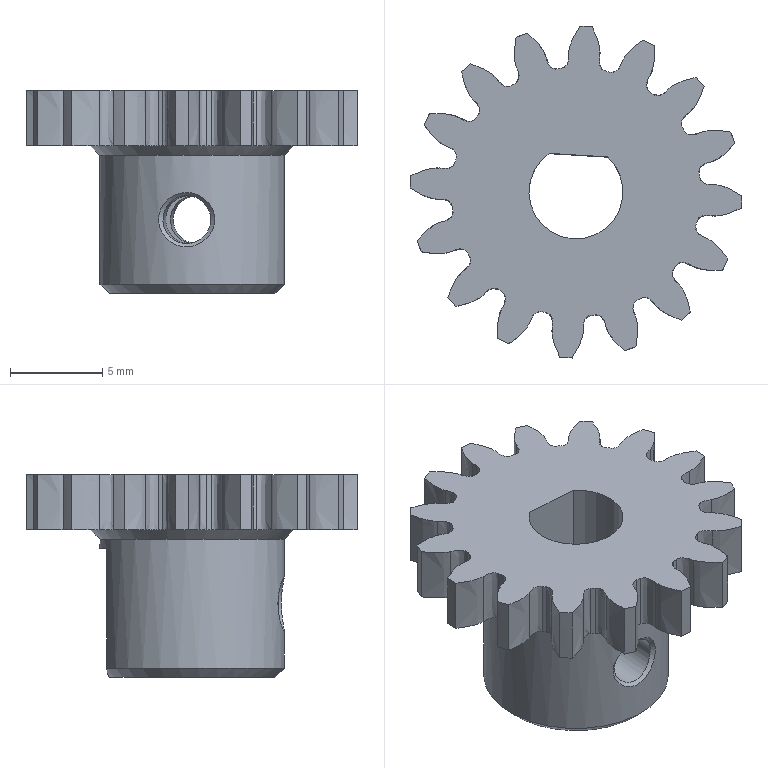Component | NX | DJZ_02_GEAR1 | 1 solid | 111 faces | volume 968 mm3 | other 80 | cylinder 20 | plane 7 | cone 3 | spline 1 | commonest cylinder face diameters 13.5 x16 2.6 x2 10 x1 5.1 x1